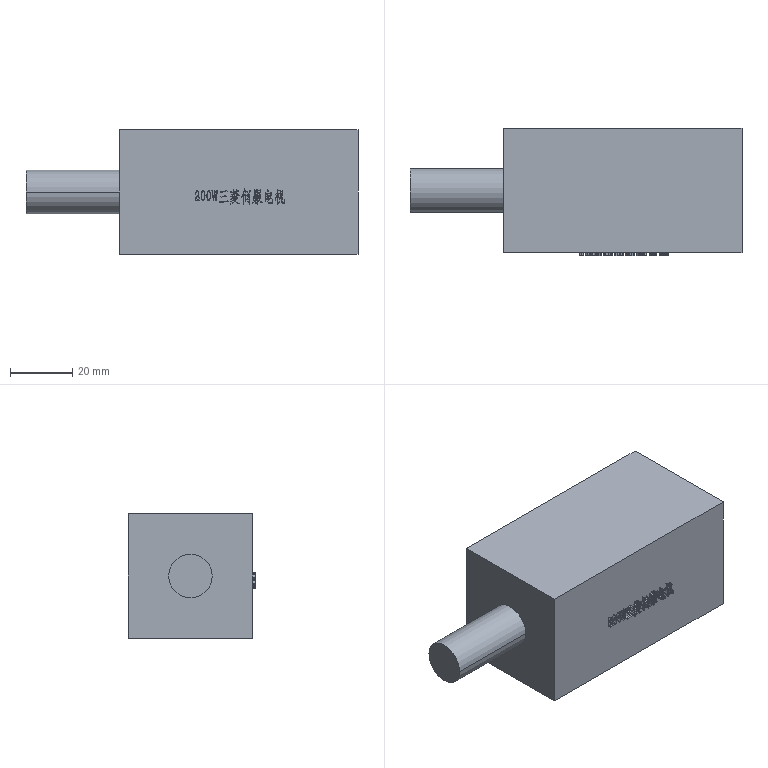Component | SolidWorks | 200WServoMotor-1 | 1 solid | 621 faces | box 106.6 x 41 x 40 mm | volume 127199 mm3 | plane 443 | spline 176 | cylinder 2 | commonest cylinder face diameters 14 x2